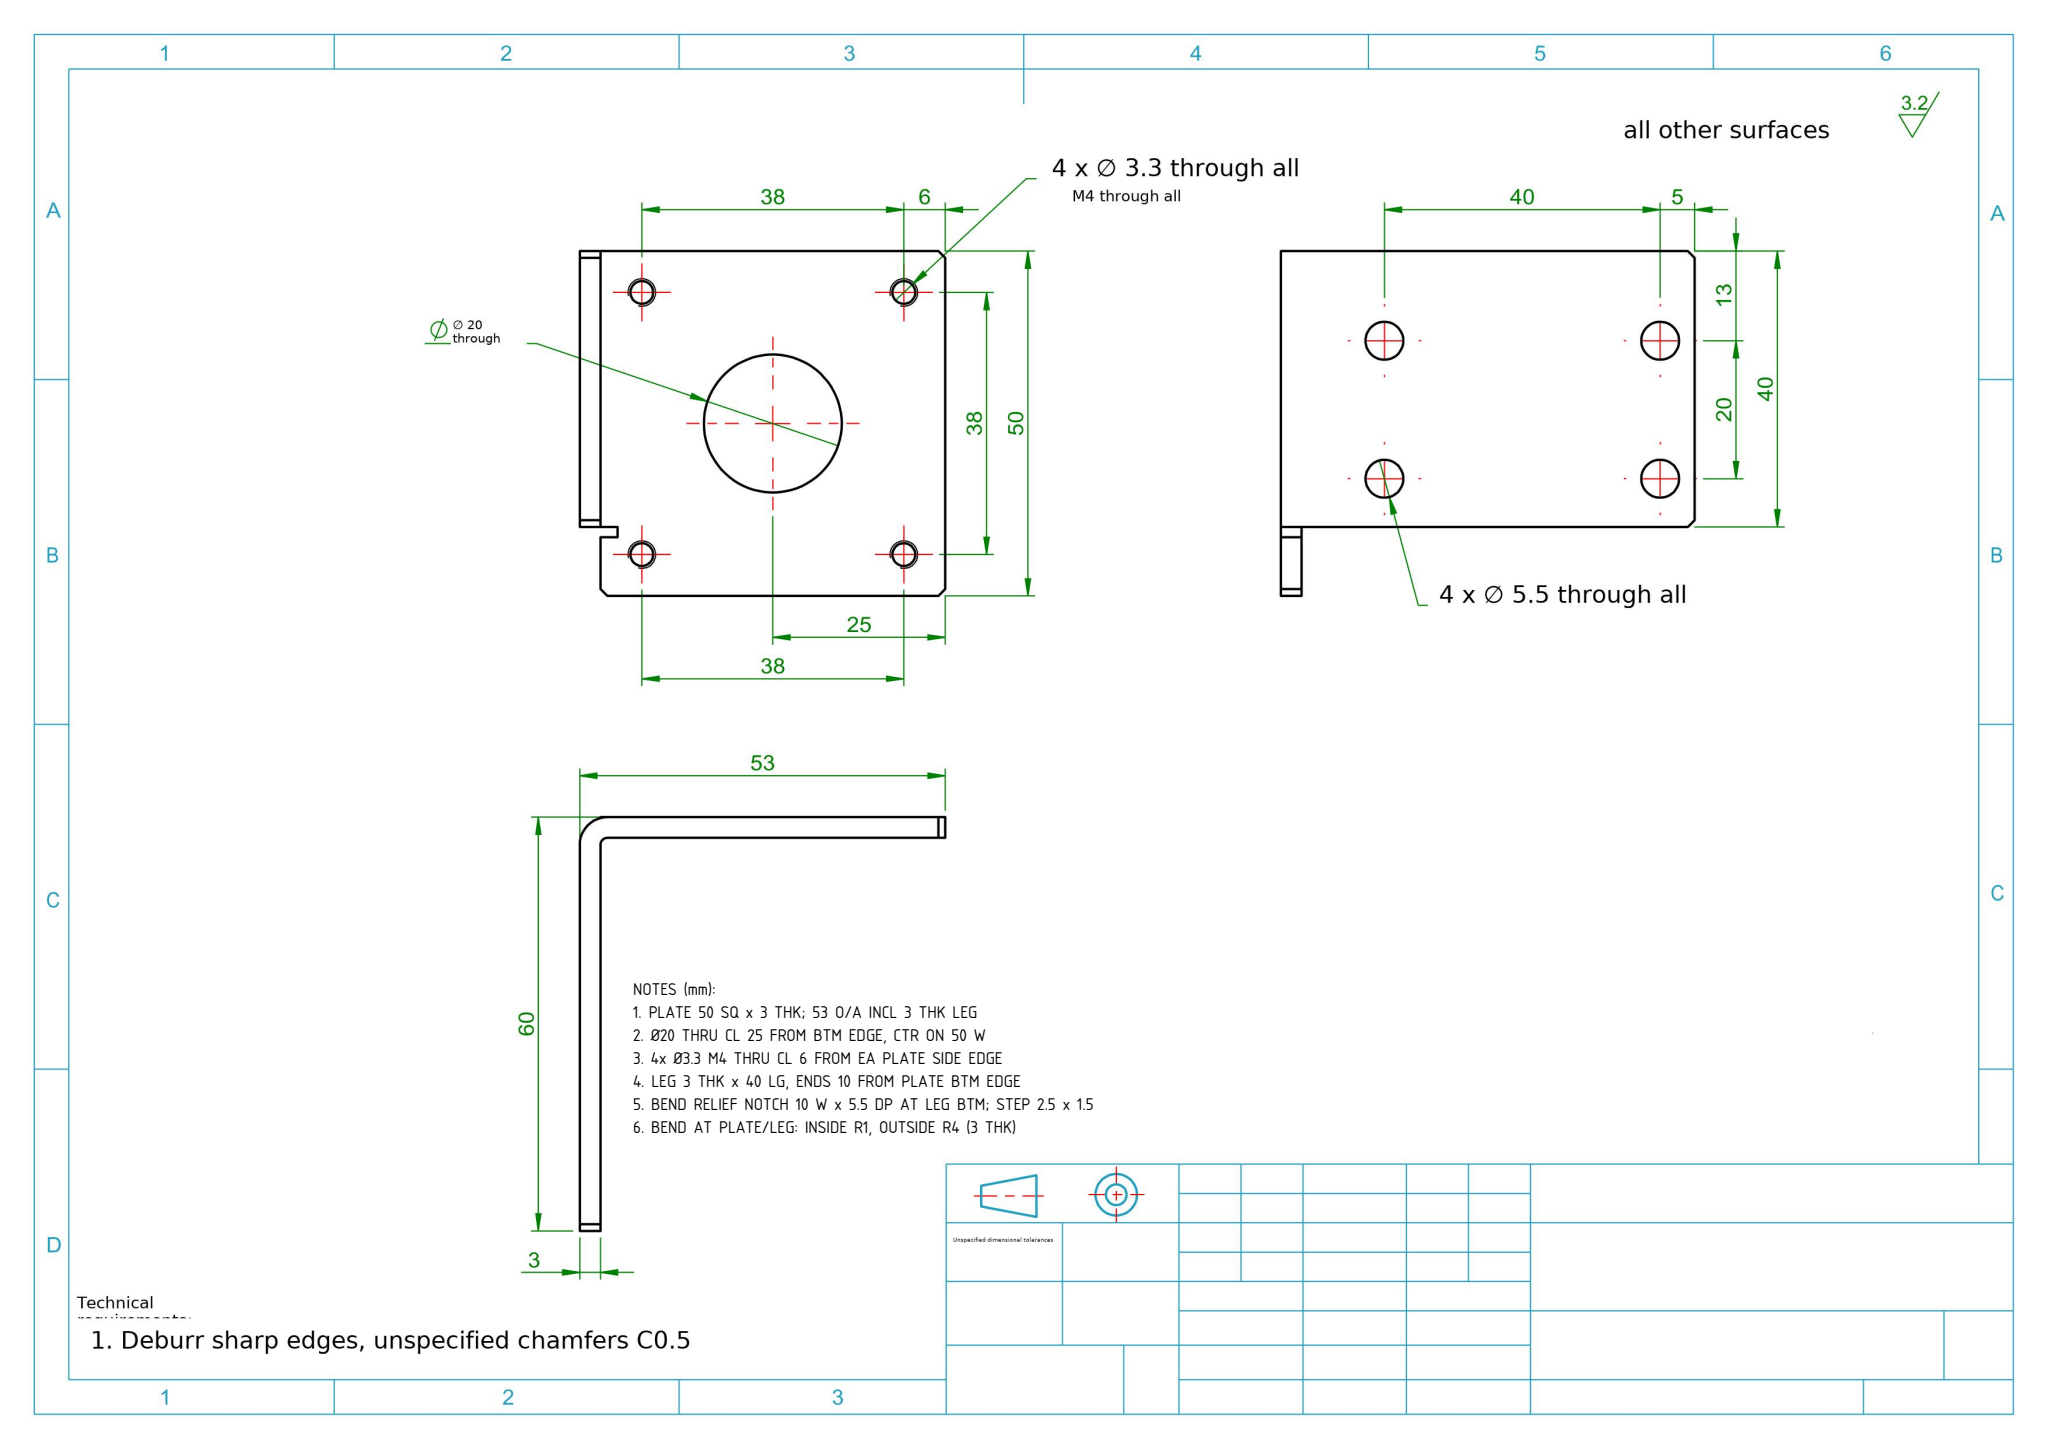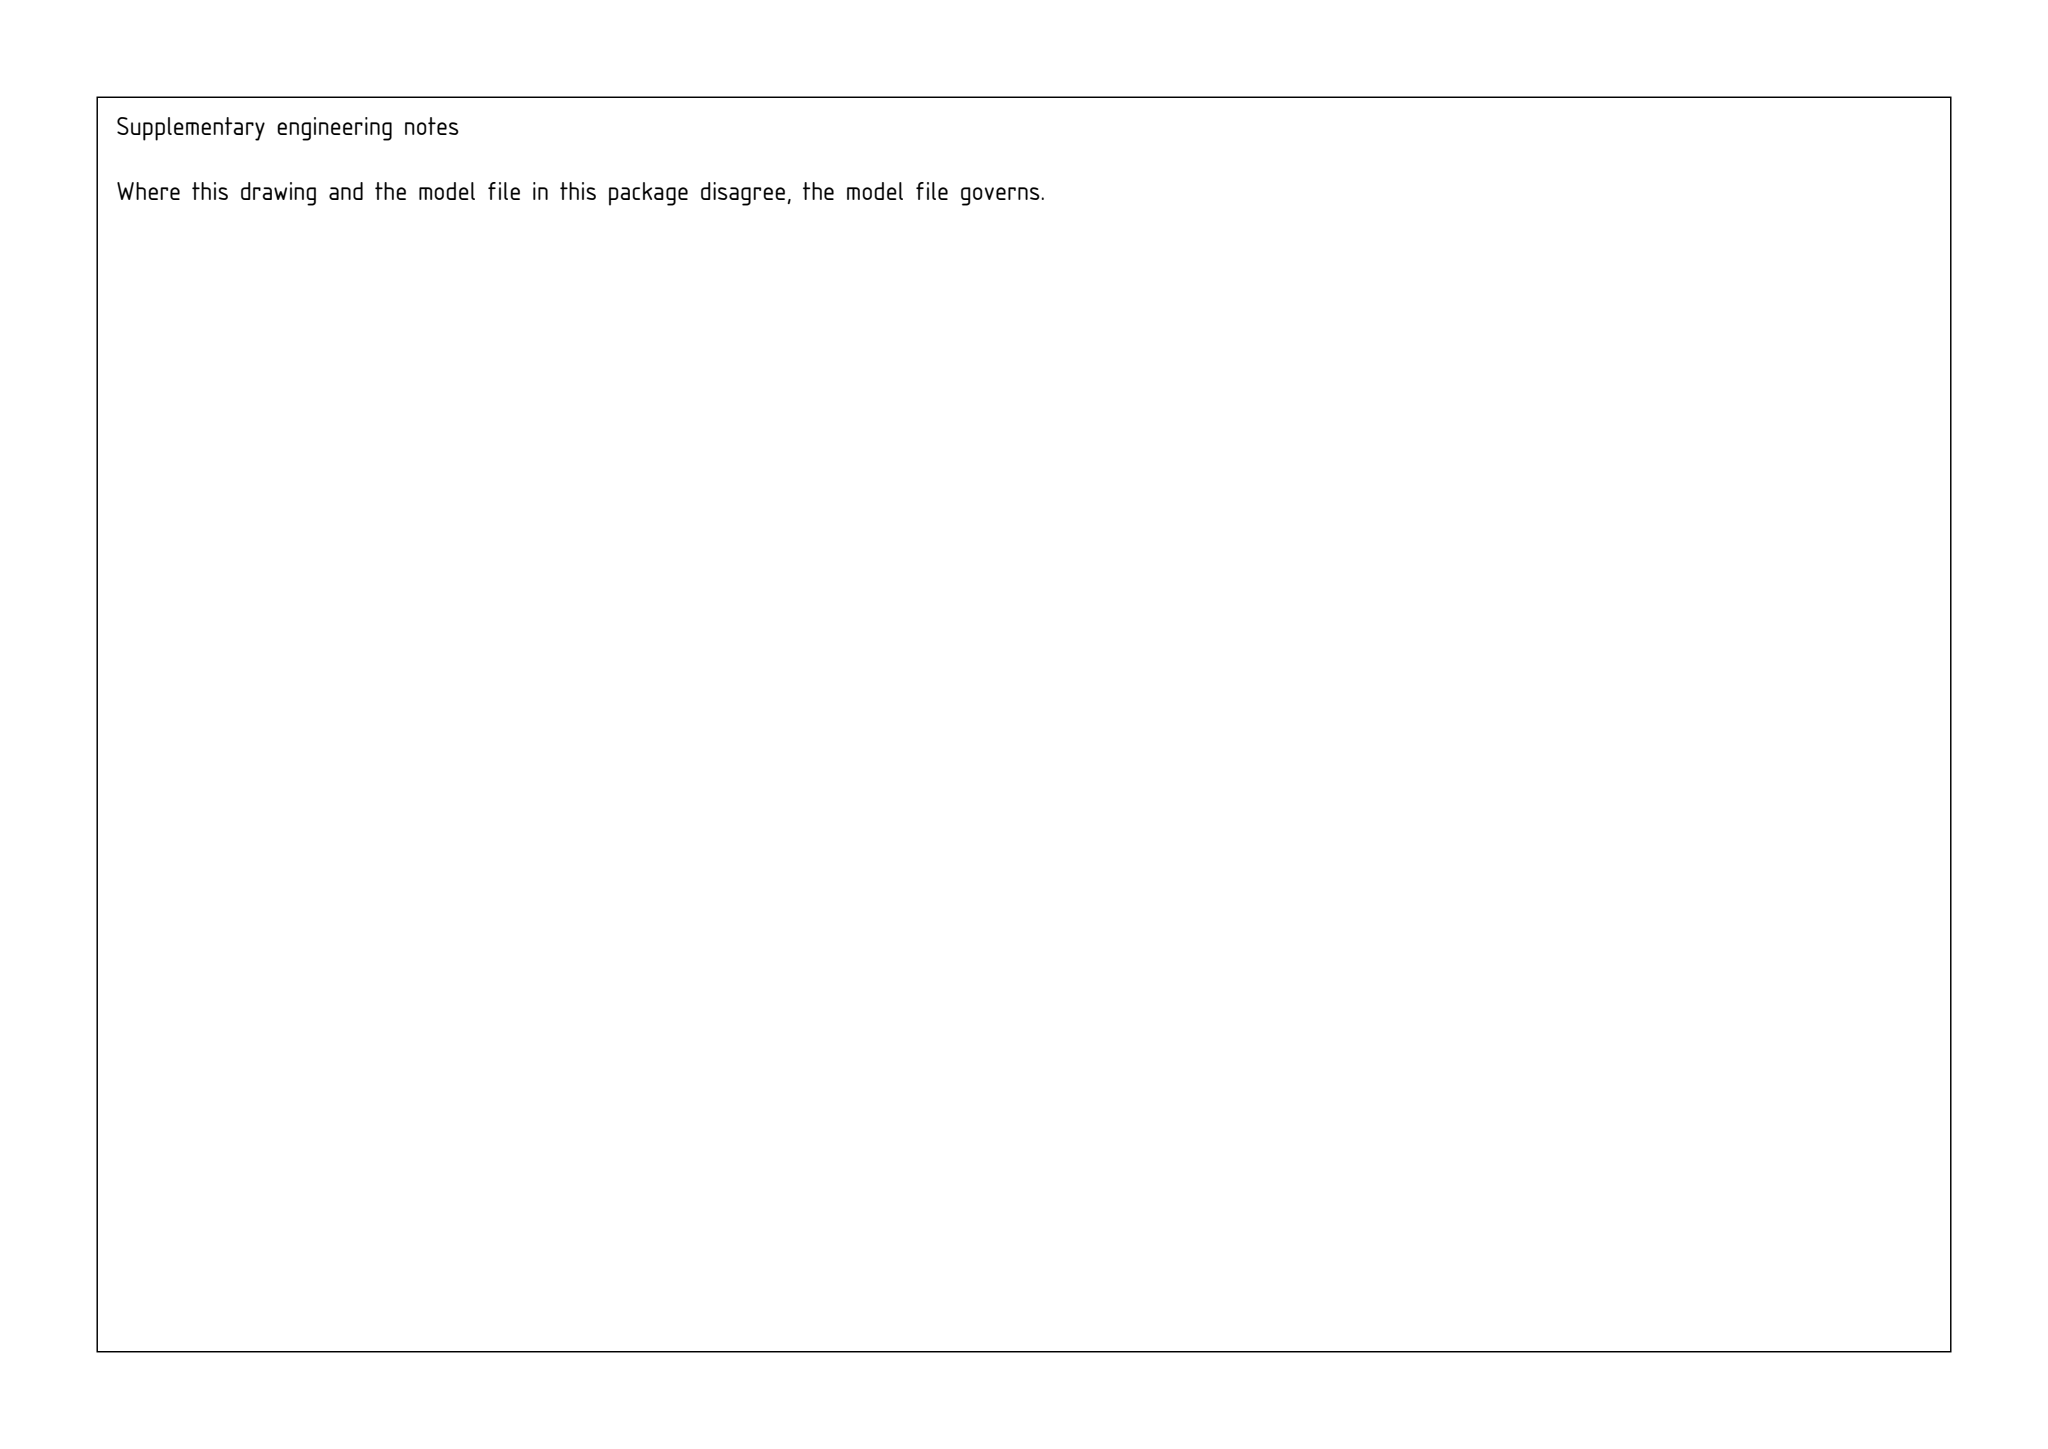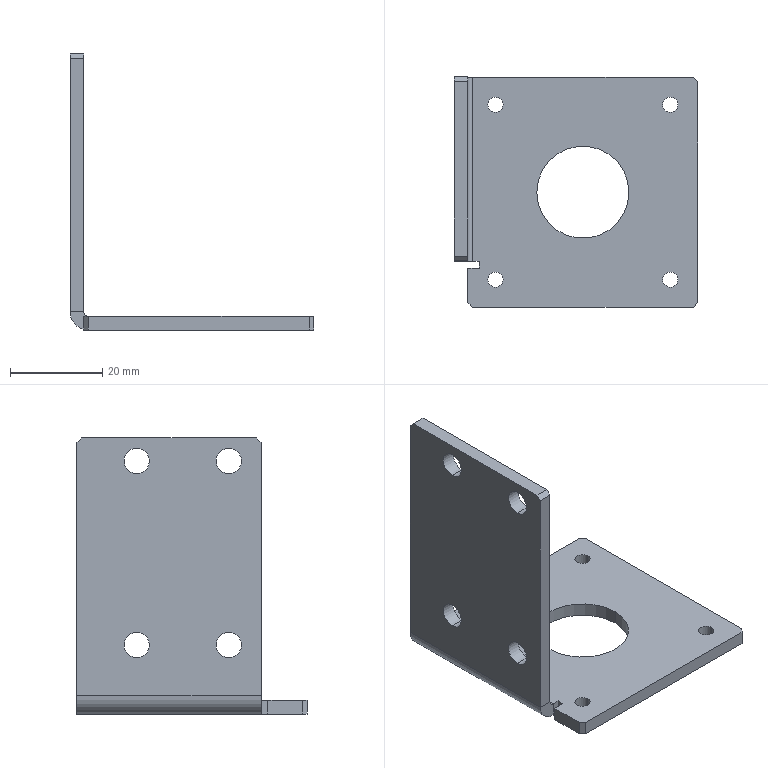Part | SolidWorks | mm | 1 solid | 41 faces | box 53 x 50 x 60 mm | volume 13222 mm3 | plane 21 | cylinder 20 | commonest cylinder face diameters 5.5 x8 3.3 x8 20 x2 8 x1 2 x1
Drawing notes:
PLATE 50 SQ x 3 THK; 53 O/A INCL 3 THK LEG | from the solid: plate faces x=3 & x=53 (50 W), y=0 & y=50, z=0 & z=3; bbox x=53
Ø20 THRU CL 25 FROM BTM EDGE, CTR ON 50 W | from the solid: Ø20 z-axis cyl at x=28, y=25; y faces 0 and 50
4x Ø3.3 M4 THRU CL 6 FROM EA PLATE SIDE EDGE | from the solid: Ø3.3 holes at x=9 & 47; plate edges x=3 and x=53
LEG 3 THK x 40 LG, ENDS 10 FROM PLATE BTM EDGE | from the solid: leg x=0-3 spans y=10 to y=50 (40 lg); plate edge y=0
BEND RELIEF NOTCH 10 W x 5.5 DP AT LEG BTM; STEP 2.5 x 1.5 | from the solid: planes y=10.0 and x=5.5 from outer face x=0; step planes x=5.5 & y=8.5
BEND AT PLATE/LEG: INSIDE R1, OUTSIDE R4 (3 THK) | from the solid: Cylinders dia 2.0 and 8.0, axis Y, at (x=4, z=4), length 40 = inner R1 / outer R4 bend